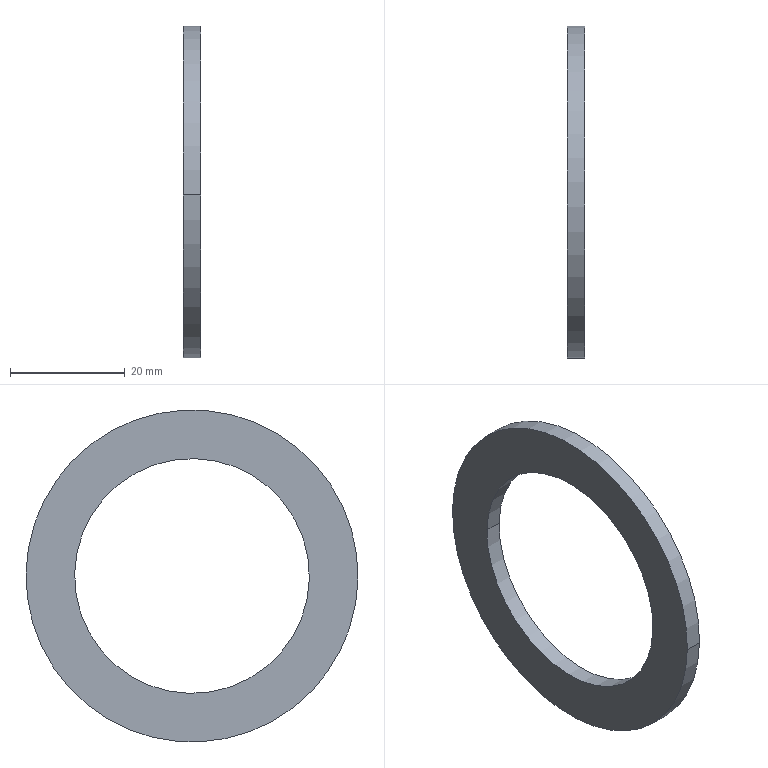Component | SolidWorks | 216InnerTubeAssembly-1_AdjustingShim-1 | 1 solid | 6 faces | box 3 x 58 x 58 mm | volume 3965 mm3 | cylinder 4 | plane 2 | commonest cylinder face diameters 41 x2 58 x2 | material Alloy Steel
build123d program:
from build123d import *

# Parameters (mm, degrees)
MODEL_W = 3
MODEL_H = 8.5


with BuildPart() as part:
    # Model → Revolve1 (revolve)
    with BuildSketch(Plane.XY, mode=Mode.PRIVATE) as revolve1_sk:
        with Locations((-1.474, 24.75)):
            Rectangle(MODEL_W, MODEL_H)
    revolve(revolve1_sk.sketch.rotate(Axis((-11.5, 0, 0), (1, 0, 0)), 180), axis=Axis((-11.5, 0, 0), (1, 0, 0)))


solid = part.part

# Placed as in the assembly
solid = solid.moved(Location((756.553, 0, 0), (0, 0, 0)))
STEP:
#1=COLOUR_RGB('',0.7922,0.8196,0.9333);
#2=FILL_AREA_STYLE_COLOUR('',#1);
#3=FILL_AREA_STYLE('',(#2));
#4=SURFACE_STYLE_FILL_AREA(#3);
#5=SURFACE_SIDE_STYLE('',(#4));
#6=SURFACE_STYLE_USAGE(.BOTH.,#5);
#7=PRESENTATION_STYLE_ASSIGNMENT((#6));
#8=CARTESIAN_POINT('',(29.787,0.807,0.01449));
#9=VERTEX_POINT('',#8);
#10=CARTESIAN_POINT('',(29.787,-0.807,-0.01449));
#11=VERTEX_POINT('',#10);
#12=CARTESIAN_POINT('',(29.787,-0.,0.));
#13=DIRECTION('',(-1.,-0.,0.));
#14=DIRECTION('',(0.,-0.9998,-0.01796));
#15=AXIS2_PLACEMENT_3D('',#12,#13,#14);
#16=CIRCLE('',#15,0.8071);
#17=EDGE_CURVE('',#9,#11,#16,.T.);
#18=ORIENTED_EDGE('',*,*,#17,.F.);
#19=CARTESIAN_POINT('',(29.668,0.807,0.01449));
#20=VERTEX_POINT('',#19);
#21=CARTESIAN_POINT('',(29.333,0.807,0.01449));
#22=DIRECTION('',(-1.,-0.,0.));
#23=VECTOR('',#22,39.37);
#24=LINE('',#21,#23);
#25=EDGE_CURVE('',#9,#20,#24,.T.);
#26=ORIENTED_EDGE('',*,*,#25,.T.);
#27=CARTESIAN_POINT('',(29.668,-0.807,-0.01449));
#28=VERTEX_POINT('',#27);
#29=CARTESIAN_POINT('',(29.668,-0.,0.));
#30=DIRECTION('',(-1.,-0.,0.));
#31=DIRECTION('',(0.,-0.9998,-0.01796));
#32=AXIS2_PLACEMENT_3D('',#29,#30,#31);
#33=CIRCLE('',#32,0.8071);
#34=EDGE_CURVE('',#20,#28,#33,.T.);
#35=ORIENTED_EDGE('',*,*,#34,.T.);
#36=CARTESIAN_POINT('',(29.333,-0.807,-0.01449));
#37=DIRECTION('',(-1.,-0.,0.));
#38=VECTOR('',#37,39.37);
#39=LINE('',#36,#38);
#40=EDGE_CURVE('',#11,#28,#39,.T.);
#41=ORIENTED_EDGE('',*,*,#40,.F.);
#42=EDGE_LOOP('',(#18,#26,#35,#41));
#43=FACE_OUTER_BOUND('',#42,.T.);
#44=CARTESIAN_POINT('',(29.333,-0.,0.));
#45=DIRECTION('',(-1.,-0.,0.));
#46=DIRECTION('',(0.,-0.9998,-0.01796));
#47=AXIS2_PLACEMENT_3D('',#44,#45,#46);
#48=CYLINDRICAL_SURFACE('',#47,0.8071);
#49=ADVANCED_FACE('',(#43),#48,.F.);
#50=CARTESIAN_POINT('',(29.787,-1.142,-0.0205));
#51=VERTEX_POINT('',#50);
#52=CARTESIAN_POINT('',(29.787,1.142,0.0205));
#53=VERTEX_POINT('',#52);
#54=CARTESIAN_POINT('',(29.787,-0.,0.));
#55=DIRECTION('',(-1.,-0.,0.));
#56=DIRECTION('',(0.,-0.9998,-0.01796));
#57=AXIS2_PLACEMENT_3D('',#54,#55,#56);
#58=CIRCLE('',#57,1.142);
#59=EDGE_CURVE('',#51,#53,#58,.T.);
#60=ORIENTED_EDGE('',*,*,#59,.T.);
#61=CARTESIAN_POINT('',(29.668,1.142,0.0205));
#62=VERTEX_POINT('',#61);
#63=CARTESIAN_POINT('',(29.333,1.142,0.0205));
#64=DIRECTION('',(-1.,-0.,0.));
#65=VECTOR('',#64,39.37);
#66=LINE('',#63,#65);
#67=EDGE_CURVE('',#53,#62,#66,.T.);
#68=ORIENTED_EDGE('',*,*,#67,.T.);
#69=CARTESIAN_POINT('',(29.668,-1.142,-0.0205));
#70=VERTEX_POINT('',#69);
#71=CARTESIAN_POINT('',(29.668,-0.,0.));
#72=DIRECTION('',(-1.,-0.,0.));
#73=DIRECTION('',(0.,-0.9998,-0.01796));
#74=AXIS2_PLACEMENT_3D('',#71,#72,#73);
#75=CIRCLE('',#74,1.142);
#76=EDGE_CURVE('',#70,#62,#75,.T.);
#77=ORIENTED_EDGE('',*,*,#76,.F.);
#78=CARTESIAN_POINT('',(29.333,-1.142,-0.0205));
#79=DIRECTION('',(-1.,-0.,0.));
#80=VECTOR('',#79,39.37);
#81=LINE('',#78,#80);
#82=EDGE_CURVE('',#51,#70,#81,.T.);
#83=ORIENTED_EDGE('',*,*,#82,.F.);
#84=EDGE_LOOP('',(#60,#68,#77,#83));
#85=FACE_OUTER_BOUND('',#84,.T.);
#86=CARTESIAN_POINT('',(29.333,-0.,0.));
#87=DIRECTION('',(-1.,-0.,0.));
#88=DIRECTION('',(0.,-0.9998,-0.01796));
#89=AXIS2_PLACEMENT_3D('',#86,#87,#88);
#90=CYLINDRICAL_SURFACE('',#89,1.142);
#91=ADVANCED_FACE('',(#85),#90,.T.);
#92=ORIENTED_EDGE('',*,*,#67,.F.);
#93=CARTESIAN_POINT('',(29.787,-0.,0.));
#94=DIRECTION('',(-1.,-0.,0.));
#95=DIRECTION('',(0.,-0.9998,-0.01796));
#96=AXIS2_PLACEMENT_3D('',#93,#94,#95);
#97=CIRCLE('',#96,1.142);
#98=EDGE_CURVE('',#53,#51,#97,.T.);
#99=ORIENTED_EDGE('',*,*,#98,.T.);
#100=ORIENTED_EDGE('',*,*,#82,.T.);
#101=CARTESIAN_POINT('',(29.668,-0.,0.));
#102=DIRECTION('',(-1.,-0.,0.));
#103=DIRECTION('',(0.,-0.9998,-0.01796));
#104=AXIS2_PLACEMENT_3D('',#101,#102,#103);
#105=CIRCLE('',#104,1.142);
#106=EDGE_CURVE('',#62,#70,#105,.T.);
#107=ORIENTED_EDGE('',*,*,#106,.F.);
#108=EDGE_LOOP('',(#92,#99,#100,#107));
#109=FACE_OUTER_BOUND('',#108,.T.);
#110=CARTESIAN_POINT('',(29.333,-0.,0.));
#111=DIRECTION('',(-1.,-0.,0.));
#112=DIRECTION('',(0.,-0.9998,-0.01796));
#113=AXIS2_PLACEMENT_3D('',#110,#111,#112);
#114=CYLINDRICAL_SURFACE('',#113,1.142);
#115=ADVANCED_FACE('',(#109),#114,.T.);
#116=CARTESIAN_POINT('',(29.668,-0.,0.));
#117=DIRECTION('',(-1.,-0.,0.));
#118=DIRECTION('',(0.,-0.9998,-0.01796));
#119=AXIS2_PLACEMENT_3D('',#116,#117,#118);
#120=CIRCLE('',#119,0.8071);
#121=EDGE_CURVE('',#28,#20,#120,.T.);
#122=ORIENTED_EDGE('',*,*,#121,.F.);
#123=ORIENTED_EDGE('',*,*,#34,.F.);
#124=EDGE_LOOP('',(#122,#123));
#125=FACE_BOUND('',#124,.T.);
#126=ORIENTED_EDGE('',*,*,#76,.T.);
#127=ORIENTED_EDGE('',*,*,#106,.T.);
#128=EDGE_LOOP('',(#126,#127));
#129=FACE_OUTER_BOUND('',#128,.T.);
#130=CARTESIAN_POINT('',(29.668,1.142,0.0205));
#131=DIRECTION('',(1.,0.,-0.));
#132=DIRECTION('',(-0.,0.9998,0.01796));
#133=AXIS2_PLACEMENT_3D('',#130,#131,#132);
#134=PLANE('',#133);
#135=ADVANCED_FACE('',(#125,#129),#134,.F.);
#136=ORIENTED_EDGE('',*,*,#25,.F.);
#137=CARTESIAN_POINT('',(29.787,-0.,0.));
#138=DIRECTION('',(-1.,-0.,0.));
#139=DIRECTION('',(0.,-0.9998,-0.01796));
#140=AXIS2_PLACEMENT_3D('',#137,#138,#139);
#141=CIRCLE('',#140,0.8071);
#142=EDGE_CURVE('',#11,#9,#141,.T.);
#143=ORIENTED_EDGE('',*,*,#142,.F.);
#144=ORIENTED_EDGE('',*,*,#40,.T.);
#145=ORIENTED_EDGE('',*,*,#121,.T.);
#146=EDGE_LOOP('',(#136,#143,#144,#145));
#147=FACE_OUTER_BOUND('',#146,.T.);
#148=CARTESIAN_POINT('',(29.333,-0.,0.));
#149=DIRECTION('',(-1.,-0.,0.));
#150=DIRECTION('',(0.,-0.9998,-0.01796));
#151=AXIS2_PLACEMENT_3D('',#148,#149,#150);
#152=CYLINDRICAL_SURFACE('',#151,0.8071);
#153=ADVANCED_FACE('',(#147),#152,.F.);
#154=ORIENTED_EDGE('',*,*,#59,.F.);
#155=ORIENTED_EDGE('',*,*,#98,.F.);
#156=EDGE_LOOP('',(#154,#155));
#157=FACE_OUTER_BOUND('',#156,.T.);
#158=ORIENTED_EDGE('',*,*,#142,.T.);
#159=ORIENTED_EDGE('',*,*,#17,.T.);
#160=EDGE_LOOP('',(#158,#159));
#161=FACE_BOUND('',#160,.T.);
#162=CARTESIAN_POINT('',(29.787,1.142,0.0205));
#163=DIRECTION('',(-1.,-0.,0.));
#164=DIRECTION('',(0.,-0.9998,-0.01796));
#165=AXIS2_PLACEMENT_3D('',#162,#163,#164);
#166=PLANE('',#165);
#167=ADVANCED_FACE('',(#157,#161),#166,.F.);
#168=CLOSED_SHELL('',(#49,#91,#115,#135,#153,#167));
#169=MANIFOLD_SOLID_BREP('',#168);
#170=STYLED_ITEM('',(#7),#169);
#171=PRESENTATION_LAYER_ASSIGNMENT('','',(#170));
#172=(LENGTH_UNIT()NAMED_UNIT(*)SI_UNIT($,.METRE.));
#173=LENGTH_MEASURE_WITH_UNIT(LENGTH_MEASURE(0.0254),#172);
#174=DIMENSIONAL_EXPONENTS(1.,0.,0.,0.,0.,0.,0.);
#175=(CONVERSION_BASED_UNIT('',#173)LENGTH_UNIT()NAMED_UNIT(#174));
#176=UNCERTAINTY_MEASURE_WITH_UNIT(LENGTH_MEASURE(0.00001),#175,'','');
#177=(NAMED_UNIT(*)PLANE_ANGLE_UNIT()SI_UNIT($,.RADIAN.));
#178=(NAMED_UNIT(*)SI_UNIT($,.STERADIAN.)SOLID_ANGLE_UNIT());
#179=(GEOMETRIC_REPRESENTATION_CONTEXT(3)GLOBAL_UNCERTAINTY_ASSIGNED_CONTEXT((#176))GLOBAL_UNIT_ASSIGNED_CONTEXT((#175,#177,#178))REPRESENTATION_CONTEXT('',''));
#180=MECHANICAL_DESIGN_GEOMETRIC_PRESENTATION_REPRESENTATION('',(#170),#179);
#181=CARTESIAN_POINT('',(0.,0.,0.));
#182=DIRECTION('',(0.,0.,1.));
#183=DIRECTION('',(1.,0.,0.));
#184=AXIS2_PLACEMENT_3D('',#181,#182,#183);
#185=(LENGTH_UNIT()NAMED_UNIT(*)SI_UNIT($,.METRE.));
#186=LENGTH_MEASURE_WITH_UNIT(LENGTH_MEASURE(0.0254),#185);
#187=DIMENSIONAL_EXPONENTS(1.,0.,0.,0.,0.,0.,0.);
#188=(CONVERSION_BASED_UNIT('',#186)LENGTH_UNIT()NAMED_UNIT(#187));
#189=UNCERTAINTY_MEASURE_WITH_UNIT(LENGTH_MEASURE(0.00001),#188,'','');
#190=(NAMED_UNIT(*)PLANE_ANGLE_UNIT()SI_UNIT($,.RADIAN.));
#191=(NAMED_UNIT(*)SI_UNIT($,.STERADIAN.)SOLID_ANGLE_UNIT());
#192=(GEOMETRIC_REPRESENTATION_CONTEXT(3)GLOBAL_UNCERTAINTY_ASSIGNED_CONTEXT((#189))GLOBAL_UNIT_ASSIGNED_CONTEXT((#188,#190,#191))REPRESENTATION_CONTEXT('',''));
#193=ADVANCED_BREP_SHAPE_REPRESENTATION('',(#169,#184),#192);